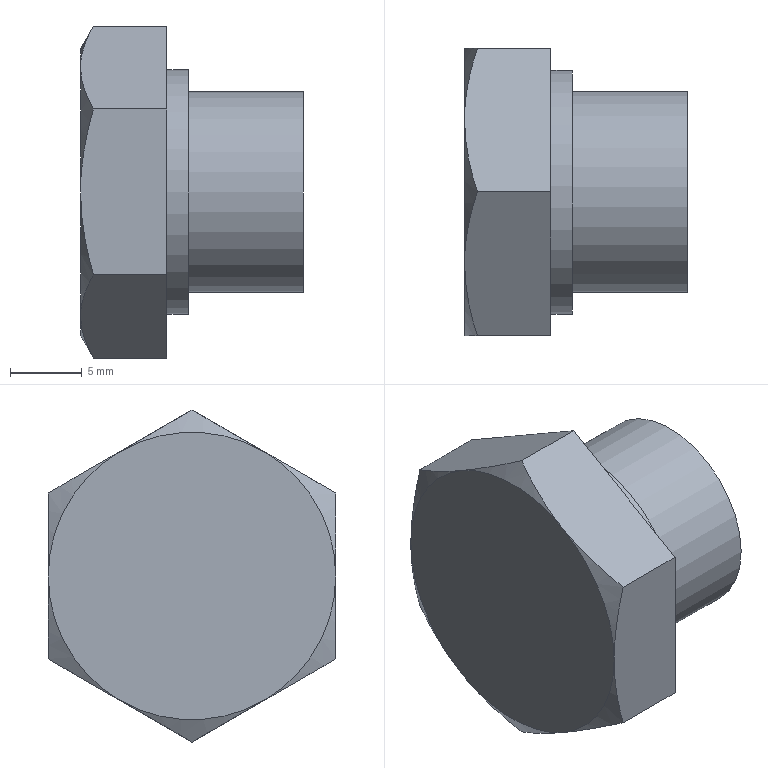Component | NX | PLUG | 1 solid | 18 faces | volume 3642 mm3 | plane 10 | cone 6 | cylinder 2 | commonest cylinder face diameters 14 x1 17 x1